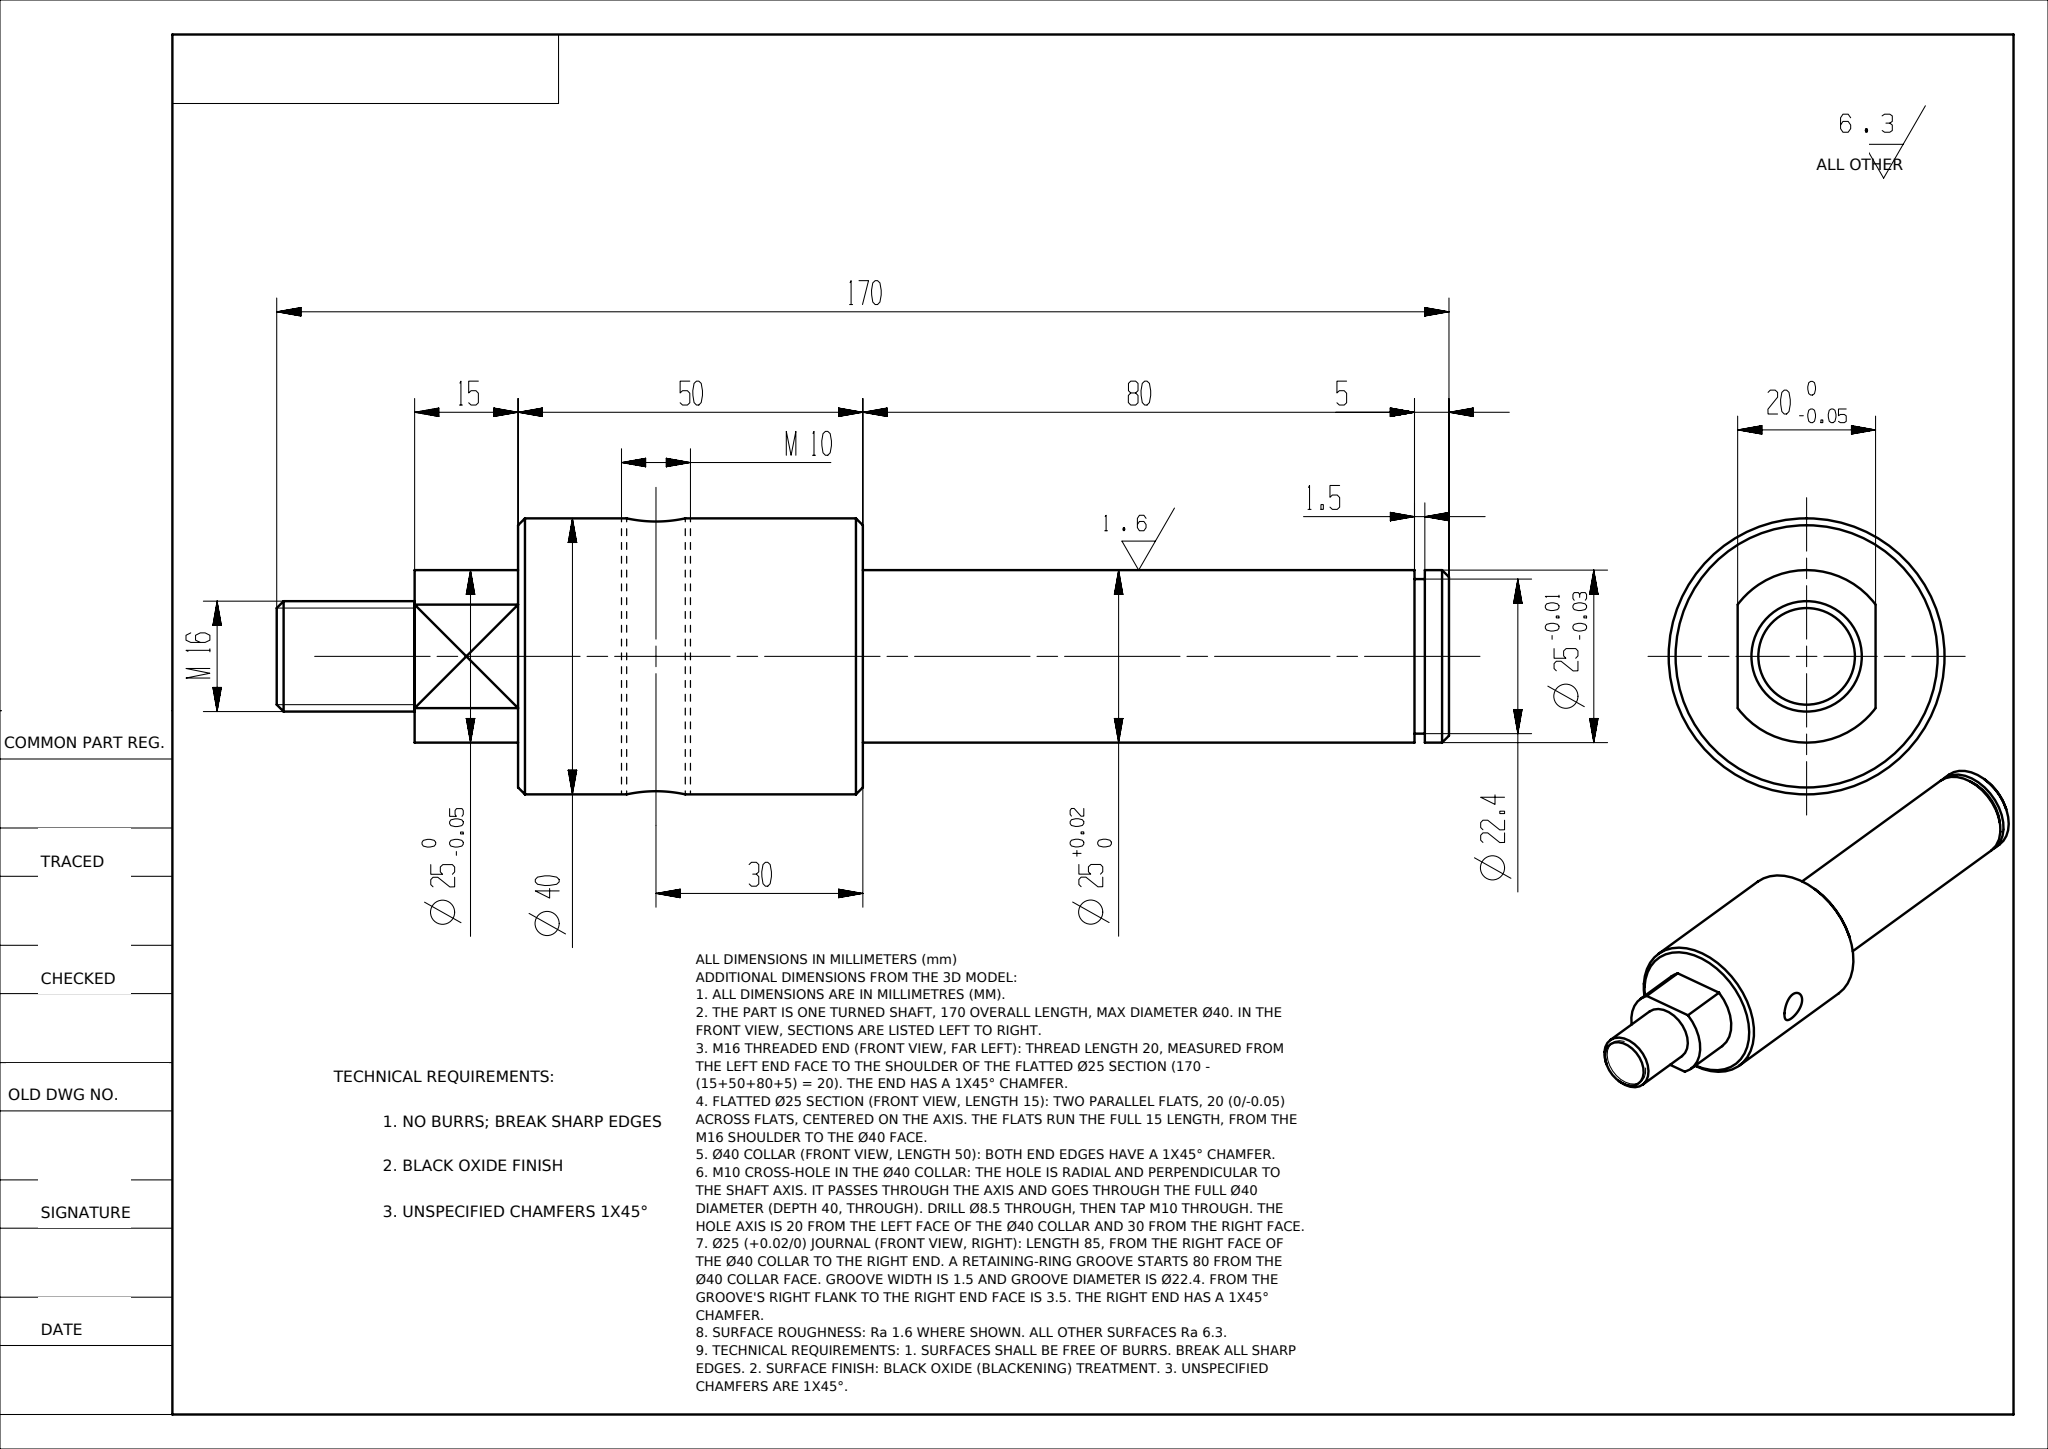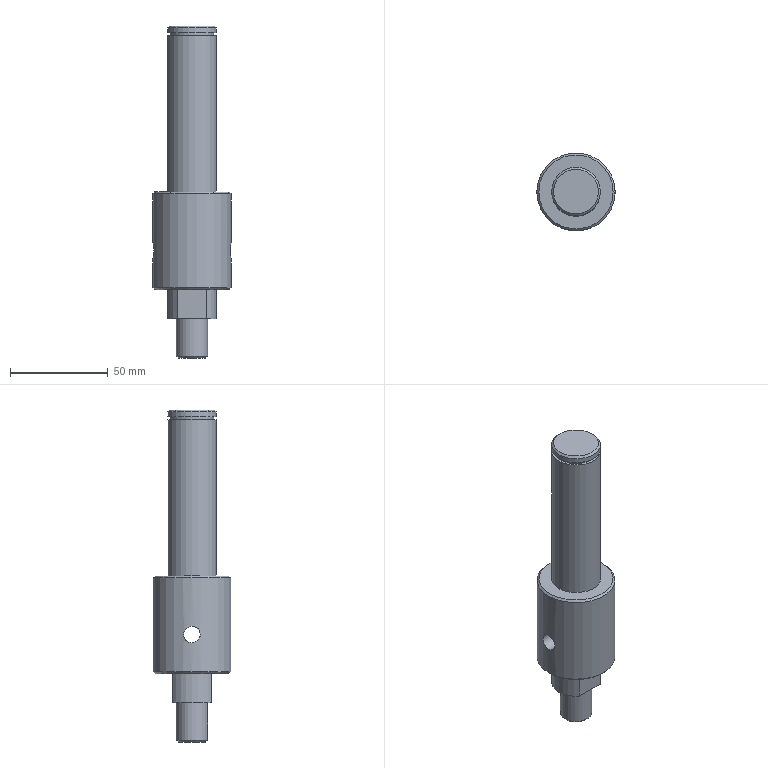Part | NX | mm | 1 solid | 21 faces | box 40 x 40 x 170 mm | volume 112586 mm3 | plane 9 | cylinder 8 | cone 4 | commonest cylinder face diameters 25 x4 40 x1 22.4 x1 16 x1 8.5 x1
STEP:
#1=CARTESIAN_POINT('',(0.,0.,0.));
#2=DIRECTION('',(0.,0.,1.));
#3=DIRECTION('',(1.,0.,0.));
#4=AXIS2_PLACEMENT_3D('',#1,#2,#3);
#5=(LENGTH_UNIT()NAMED_UNIT(*)SI_UNIT(.MILLI.,.METRE.));
#6=UNCERTAINTY_MEASURE_WITH_UNIT(LENGTH_MEASURE(0.0508),#5,'','');
#7=(NAMED_UNIT(*)PLANE_ANGLE_UNIT()SI_UNIT($,.RADIAN.));
#8=PLANE_ANGLE_MEASURE_WITH_UNIT(PLANE_ANGLE_MEASURE(0.01745),#7);
#9=DIMENSIONAL_EXPONENTS(0.,0.,0.,0.,0.,0.,0.);
#10=(CONVERSION_BASED_UNIT('',#8)NAMED_UNIT(#9)PLANE_ANGLE_UNIT());
#11=(NAMED_UNIT(*)SI_UNIT($,.STERADIAN.)SOLID_ANGLE_UNIT());
#12=(GEOMETRIC_REPRESENTATION_CONTEXT(3)GLOBAL_UNCERTAINTY_ASSIGNED_CONTEXT((#6))GLOBAL_UNIT_ASSIGNED_CONTEXT((#5,#10,#11))REPRESENTATION_CONTEXT('',''));
#13=SHAPE_REPRESENTATION('',(#4),#12);
#14=CARTESIAN_POINT('',(-7.5,10.,-15.));
#15=VERTEX_POINT('',#14);
#16=CARTESIAN_POINT('',(-7.5,10.,0.));
#17=VERTEX_POINT('',#16);
#18=CARTESIAN_POINT('',(-7.5,10.,0.));
#19=DIRECTION('',(0.,0.,1.));
#20=VECTOR('',#19,1.);
#21=LINE('',#18,#20);
#22=EDGE_CURVE('',#15,#17,#21,.T.);
#23=ORIENTED_EDGE('',*,*,#22,.F.);
#24=CARTESIAN_POINT('',(-7.5,-10.,-15.));
#25=VERTEX_POINT('',#24);
#26=CARTESIAN_POINT('',(0.,0.,-15.));
#27=DIRECTION('',(0.,0.,1.));
#28=DIRECTION('',(1.,0.,0.));
#29=AXIS2_PLACEMENT_3D('',#26,#27,#28);
#30=CIRCLE('',#29,12.5);
#31=EDGE_CURVE('',#15,#25,#30,.T.);
#32=ORIENTED_EDGE('',*,*,#31,.T.);
#33=CARTESIAN_POINT('',(-7.5,-10.,0.));
#34=VERTEX_POINT('',#33);
#35=CARTESIAN_POINT('',(-7.5,-10.,0.));
#36=DIRECTION('',(0.,0.,-1.));
#37=VECTOR('',#36,1.);
#38=LINE('',#35,#37);
#39=EDGE_CURVE('',#34,#25,#38,.T.);
#40=ORIENTED_EDGE('',*,*,#39,.F.);
#41=CARTESIAN_POINT('',(0.,0.,0.));
#42=DIRECTION('',(0.,0.,-1.));
#43=DIRECTION('',(-1.,0.,0.));
#44=AXIS2_PLACEMENT_3D('',#41,#42,#43);
#45=CIRCLE('',#44,12.5);
#46=EDGE_CURVE('',#34,#17,#45,.T.);
#47=ORIENTED_EDGE('',*,*,#46,.T.);
#48=EDGE_LOOP('',(#23,#32,#40,#47));
#49=FACE_OUTER_BOUND('',#48,.T.);
#50=CARTESIAN_POINT('',(0.,0.,0.));
#51=DIRECTION('',(0.,0.,-1.));
#52=DIRECTION('',(1.,0.,0.));
#53=AXIS2_PLACEMENT_3D('',#50,#51,#52);
#54=CYLINDRICAL_SURFACE('',#53,12.5);
#55=ADVANCED_FACE('',(#49),#54,.T.);
#56=CARTESIAN_POINT('',(12.5,0.,50.));
#57=VERTEX_POINT('',#56);
#58=CARTESIAN_POINT('',(0.,0.,50.));
#59=DIRECTION('',(0.,0.,1.));
#60=DIRECTION('',(1.,0.,0.));
#61=AXIS2_PLACEMENT_3D('',#58,#59,#60);
#62=CIRCLE('',#61,12.5);
#63=EDGE_CURVE('',#57,#57,#62,.T.);
#64=ORIENTED_EDGE('',*,*,#63,.T.);
#65=EDGE_LOOP('',(#64));
#66=FACE_BOUND('',#65,.T.);
#67=CARTESIAN_POINT('',(12.5,0.,130.));
#68=VERTEX_POINT('',#67);
#69=CARTESIAN_POINT('',(0.,0.,130.));
#70=DIRECTION('',(0.,0.,-1.));
#71=DIRECTION('',(1.,0.,0.));
#72=AXIS2_PLACEMENT_3D('',#69,#70,#71);
#73=CIRCLE('',#72,12.5);
#74=EDGE_CURVE('',#68,#68,#73,.T.);
#75=ORIENTED_EDGE('',*,*,#74,.T.);
#76=EDGE_LOOP('',(#75));
#77=FACE_BOUND('',#76,.T.);
#78=CARTESIAN_POINT('',(0.,0.,40.));
#79=DIRECTION('',(0.,0.,1.));
#80=DIRECTION('',(1.,0.,0.));
#81=AXIS2_PLACEMENT_3D('',#78,#79,#80);
#82=CYLINDRICAL_SURFACE('',#81,12.5);
#83=ADVANCED_FACE('',(#66,#77),#82,.T.);
#84=CARTESIAN_POINT('',(19.,0.,50.));
#85=VERTEX_POINT('',#84);
#86=CARTESIAN_POINT('',(0.,0.,50.));
#87=DIRECTION('',(0.,0.,1.));
#88=DIRECTION('',(1.,0.,0.));
#89=AXIS2_PLACEMENT_3D('',#86,#87,#88);
#90=CIRCLE('',#89,19.);
#91=EDGE_CURVE('',#85,#85,#90,.T.);
#92=ORIENTED_EDGE('',*,*,#91,.T.);
#93=EDGE_LOOP('',(#92));
#94=FACE_BOUND('',#93,.T.);
#95=ORIENTED_EDGE('',*,*,#63,.F.);
#96=EDGE_LOOP('',(#95));
#97=FACE_BOUND('',#96,.T.);
#98=CARTESIAN_POINT('',(0.,0.,50.));
#99=DIRECTION('',(0.,0.,1.));
#100=DIRECTION('',(1.,0.,0.));
#101=AXIS2_PLACEMENT_3D('',#98,#99,#100);
#102=PLANE('',#101);
#103=ADVANCED_FACE('',(#94,#97),#102,.T.);
#104=CARTESIAN_POINT('',(-19.,0.,0.));
#105=VERTEX_POINT('',#104);
#106=CARTESIAN_POINT('',(0.,0.,0.));
#107=DIRECTION('',(0.,0.,-1.));
#108=DIRECTION('',(-1.,0.,0.));
#109=AXIS2_PLACEMENT_3D('',#106,#107,#108);
#110=CIRCLE('',#109,19.);
#111=EDGE_CURVE('',#105,#105,#110,.T.);
#112=ORIENTED_EDGE('',*,*,#111,.T.);
#113=EDGE_LOOP('',(#112));
#114=FACE_BOUND('',#113,.T.);
#115=CARTESIAN_POINT('',(7.5,10.,0.));
#116=VERTEX_POINT('',#115);
#117=CARTESIAN_POINT('',(7.5,-10.,0.));
#118=VERTEX_POINT('',#117);
#119=CARTESIAN_POINT('',(0.,0.,0.));
#120=DIRECTION('',(0.,0.,-1.));
#121=DIRECTION('',(-1.,0.,0.));
#122=AXIS2_PLACEMENT_3D('',#119,#120,#121);
#123=CIRCLE('',#122,12.5);
#124=EDGE_CURVE('',#116,#118,#123,.T.);
#125=ORIENTED_EDGE('',*,*,#124,.F.);
#126=CARTESIAN_POINT('',(13.5,10.,0.));
#127=DIRECTION('',(-1.,0.,0.));
#128=VECTOR('',#127,1.);
#129=LINE('',#126,#128);
#130=EDGE_CURVE('',#116,#17,#129,.T.);
#131=ORIENTED_EDGE('',*,*,#130,.T.);
#132=ORIENTED_EDGE('',*,*,#46,.F.);
#133=CARTESIAN_POINT('',(-14.,-10.,0.));
#134=DIRECTION('',(1.,0.,0.));
#135=VECTOR('',#134,1.);
#136=LINE('',#133,#135);
#137=EDGE_CURVE('',#34,#118,#136,.T.);
#138=ORIENTED_EDGE('',*,*,#137,.T.);
#139=EDGE_LOOP('',(#125,#131,#132,#138));
#140=FACE_BOUND('',#139,.T.);
#141=CARTESIAN_POINT('',(0.,0.,0.));
#142=DIRECTION('',(0.,0.,-1.));
#143=DIRECTION('',(-1.,0.,0.));
#144=AXIS2_PLACEMENT_3D('',#141,#142,#143);
#145=PLANE('',#144);
#146=ADVANCED_FACE('',(#114,#140),#145,.T.);
#147=CARTESIAN_POINT('',(20.,0.,15.75));
#148=VERTEX_POINT('',#147);
#149=CARTESIAN_POINT('',(20.,0.,15.75));
#150=CARTESIAN_POINT('',(20.,0.4698,15.75));
#151=CARTESIAN_POINT('',(19.983,0.946,15.83));
#152=CARTESIAN_POINT('',(19.952,1.389,15.983));
#153=CARTESIAN_POINT('',(19.921,1.832,16.137));
#154=CARTESIAN_POINT('',(19.876,2.254,16.367));
#155=CARTESIAN_POINT('',(19.827,2.621,16.655));
#156=CARTESIAN_POINT('',(19.778,2.994,16.947));
#157=CARTESIAN_POINT('',(19.724,3.321,17.306));
#158=CARTESIAN_POINT('',(19.678,3.577,17.705));
#159=CARTESIAN_POINT('',(19.631,3.835,18.108));
#160=CARTESIAN_POINT('',(19.591,4.028,18.562));
#161=CARTESIAN_POINT('',(19.567,4.138,19.029));
#162=CARTESIAN_POINT('',(19.544,4.246,19.49));
#163=CARTESIAN_POINT('',(19.538,4.276,19.976));
#164=CARTESIAN_POINT('',(19.548,4.226,20.447));
#165=CARTESIAN_POINT('',(19.559,4.177,20.91));
#166=CARTESIAN_POINT('',(19.587,4.05,21.371));
#167=CARTESIAN_POINT('',(19.625,3.854,21.791));
#168=CARTESIAN_POINT('',(19.664,3.657,22.215));
#169=CARTESIAN_POINT('',(19.714,3.386,22.611));
#170=CARTESIAN_POINT('',(19.764,3.062,22.947));
#171=CARTESIAN_POINT('',(19.815,2.732,23.29));
#172=CARTESIAN_POINT('',(19.867,2.339,23.581));
#173=CARTESIAN_POINT('',(19.908,1.913,23.795));
#174=CARTESIAN_POINT('',(19.949,1.486,24.01));
#175=CARTESIAN_POINT('',(19.98,1.015,24.155));
#176=CARTESIAN_POINT('',(19.993,0.5393,24.216));
#177=CARTESIAN_POINT('',(20.005,0.07279,24.275));
#178=CARTESIAN_POINT('',(20.001,-0.411,24.256));
#179=CARTESIAN_POINT('',(19.981,-0.8711,24.16));
#180=CARTESIAN_POINT('',(19.961,-1.327,24.064));
#181=CARTESIAN_POINT('',(19.925,-1.771,23.891));
#182=CARTESIAN_POINT('',(19.882,-2.17,23.654));
#183=CARTESIAN_POINT('',(19.838,-2.574,23.414));
#184=CARTESIAN_POINT('',(19.785,-2.942,23.103));
#185=CARTESIAN_POINT('',(19.735,-3.245,22.744));
#186=CARTESIAN_POINT('',(19.684,-3.554,22.379));
#187=CARTESIAN_POINT('',(19.636,-3.803,21.956));
#188=CARTESIAN_POINT('',(19.601,-3.973,21.508));
#189=CARTESIAN_POINT('',(19.567,-4.142,21.063));
#190=CARTESIAN_POINT('',(19.546,-4.237,20.581));
#191=CARTESIAN_POINT('',(19.543,-4.249,20.103));
#192=CARTESIAN_POINT('',(19.541,-4.26,19.636));
#193=CARTESIAN_POINT('',(19.556,-4.192,19.16));
#194=CARTESIAN_POINT('',(19.585,-4.051,18.715));
#195=CARTESIAN_POINT('',(19.615,-3.91,18.271));
#196=CARTESIAN_POINT('',(19.658,-3.693,17.846));
#197=CARTESIAN_POINT('',(19.706,-3.417,17.473));
#198=CARTESIAN_POINT('',(19.755,-3.136,17.093));
#199=CARTESIAN_POINT('',(19.809,-2.787,16.756));
#200=CARTESIAN_POINT('',(19.856,-2.396,16.49));
#201=CARTESIAN_POINT('',(19.904,-2.001,16.22));
#202=CARTESIAN_POINT('',(19.945,-1.552,16.015));
#203=CARTESIAN_POINT('',(19.97,-1.088,15.892));
#204=CARTESIAN_POINT('',(19.99,-0.7349,15.798));
#205=CARTESIAN_POINT('',(20.,-0.3659,15.75));
#206=CARTESIAN_POINT('',(20.,0.,15.75));
#207=B_SPLINE_CURVE_WITH_KNOTS('',3,(#149,#150,#151,#152,#153,#154,#155,#156,#157,#158,#159,#160,#161,#162,#163,#164,#165,#166,#167,#168,#169,#170,#171,#172,#173,#174,#175,#176,#177,#178,#179,#180,#181,#182,#183,#184,#185,#186,#187,#188,#189,#190,#191,#192,#193,#194,#195,#196,#197,#198,#199,#200,#201,#202,#203,#204,#205,#206),.UNSPECIFIED.,.T.,.F.,(1,3,3,3,3,3,3,3,3,3,3,3,3,3,3,3,3,3,3,3,3,1),(-0.04096,0.,0.05289,0.1057,0.1593,0.2135,0.2668,0.3192,0.372,0.4259,0.4799,0.5329,0.5853,0.6384,0.6925,0.7463,0.7989,0.8514,0.9049,0.959,1.,1.053),.UNSPECIFIED.);
#208=EDGE_CURVE('',#148,#148,#207,.T.);
#209=ORIENTED_EDGE('',*,*,#208,.F.);
#210=EDGE_LOOP('',(#209));
#211=FACE_BOUND('',#210,.T.);
#212=CARTESIAN_POINT('',(-20.,0.,24.25));
#213=VERTEX_POINT('',#212);
#214=CARTESIAN_POINT('',(-20.,0.,24.25));
#215=CARTESIAN_POINT('',(-20.,0.4698,24.25));
#216=CARTESIAN_POINT('',(-19.983,0.946,24.17));
#217=CARTESIAN_POINT('',(-19.952,1.389,24.017));
#218=CARTESIAN_POINT('',(-19.921,1.832,23.863));
#219=CARTESIAN_POINT('',(-19.876,2.254,23.633));
#220=CARTESIAN_POINT('',(-19.827,2.621,23.345));
#221=CARTESIAN_POINT('',(-19.778,2.994,23.053));
#222=CARTESIAN_POINT('',(-19.724,3.321,22.694));
#223=CARTESIAN_POINT('',(-19.678,3.577,22.295));
#224=CARTESIAN_POINT('',(-19.631,3.835,21.892));
#225=CARTESIAN_POINT('',(-19.591,4.028,21.438));
#226=CARTESIAN_POINT('',(-19.567,4.138,20.971));
#227=CARTESIAN_POINT('',(-19.544,4.246,20.51));
#228=CARTESIAN_POINT('',(-19.538,4.276,20.024));
#229=CARTESIAN_POINT('',(-19.548,4.226,19.553));
#230=CARTESIAN_POINT('',(-19.559,4.177,19.09));
#231=CARTESIAN_POINT('',(-19.587,4.05,18.629));
#232=CARTESIAN_POINT('',(-19.625,3.854,18.209));
#233=CARTESIAN_POINT('',(-19.664,3.657,17.785));
#234=CARTESIAN_POINT('',(-19.714,3.386,17.389));
#235=CARTESIAN_POINT('',(-19.764,3.062,17.053));
#236=CARTESIAN_POINT('',(-19.815,2.732,16.71));
#237=CARTESIAN_POINT('',(-19.867,2.339,16.419));
#238=CARTESIAN_POINT('',(-19.908,1.913,16.205));
#239=CARTESIAN_POINT('',(-19.949,1.486,15.99));
#240=CARTESIAN_POINT('',(-19.98,1.015,15.845));
#241=CARTESIAN_POINT('',(-19.993,0.5393,15.784));
#242=CARTESIAN_POINT('',(-20.005,0.07279,15.725));
#243=CARTESIAN_POINT('',(-20.001,-0.411,15.744));
#244=CARTESIAN_POINT('',(-19.981,-0.8711,15.84));
#245=CARTESIAN_POINT('',(-19.961,-1.327,15.936));
#246=CARTESIAN_POINT('',(-19.925,-1.771,16.109));
#247=CARTESIAN_POINT('',(-19.882,-2.17,16.346));
#248=CARTESIAN_POINT('',(-19.838,-2.574,16.586));
#249=CARTESIAN_POINT('',(-19.785,-2.942,16.897));
#250=CARTESIAN_POINT('',(-19.735,-3.245,17.256));
#251=CARTESIAN_POINT('',(-19.684,-3.554,17.621));
#252=CARTESIAN_POINT('',(-19.636,-3.803,18.044));
#253=CARTESIAN_POINT('',(-19.601,-3.973,18.492));
#254=CARTESIAN_POINT('',(-19.567,-4.142,18.937));
#255=CARTESIAN_POINT('',(-19.546,-4.237,19.419));
#256=CARTESIAN_POINT('',(-19.543,-4.249,19.897));
#257=CARTESIAN_POINT('',(-19.541,-4.26,20.364));
#258=CARTESIAN_POINT('',(-19.556,-4.192,20.84));
#259=CARTESIAN_POINT('',(-19.585,-4.051,21.285));
#260=CARTESIAN_POINT('',(-19.615,-3.91,21.729));
#261=CARTESIAN_POINT('',(-19.658,-3.693,22.154));
#262=CARTESIAN_POINT('',(-19.706,-3.417,22.527));
#263=CARTESIAN_POINT('',(-19.755,-3.136,22.907));
#264=CARTESIAN_POINT('',(-19.809,-2.787,23.244));
#265=CARTESIAN_POINT('',(-19.856,-2.396,23.51));
#266=CARTESIAN_POINT('',(-19.904,-2.001,23.78));
#267=CARTESIAN_POINT('',(-19.945,-1.552,23.985));
#268=CARTESIAN_POINT('',(-19.97,-1.088,24.108));
#269=CARTESIAN_POINT('',(-19.99,-0.7349,24.202));
#270=CARTESIAN_POINT('',(-20.,-0.3659,24.25));
#271=CARTESIAN_POINT('',(-20.,0.,24.25));
#272=B_SPLINE_CURVE_WITH_KNOTS('',3,(#214,#215,#216,#217,#218,#219,#220,#221,#222,#223,#224,#225,#226,#227,#228,#229,#230,#231,#232,#233,#234,#235,#236,#237,#238,#239,#240,#241,#242,#243,#244,#245,#246,#247,#248,#249,#250,#251,#252,#253,#254,#255,#256,#257,#258,#259,#260,#261,#262,#263,#264,#265,#266,#267,#268,#269,#270,#271),.UNSPECIFIED.,.T.,.F.,(1,3,3,3,3,3,3,3,3,3,3,3,3,3,3,3,3,3,3,3,3,1),(-0.04096,0.,0.05289,0.1057,0.1593,0.2135,0.2668,0.3192,0.372,0.4259,0.4799,0.5329,0.5853,0.6384,0.6925,0.7463,0.7989,0.8514,0.9049,0.959,1.,1.053),.UNSPECIFIED.);
#273=EDGE_CURVE('',#213,#213,#272,.T.);
#274=ORIENTED_EDGE('',*,*,#273,.F.);
#275=EDGE_LOOP('',(#274));
#276=FACE_BOUND('',#275,.T.);
#277=CARTESIAN_POINT('',(-20.,0.,49.));
#278=VERTEX_POINT('',#277);
#279=CARTESIAN_POINT('',(0.,0.,49.));
#280=DIRECTION('',(0.,0.,-1.));
#281=DIRECTION('',(-1.,0.,0.));
#282=AXIS2_PLACEMENT_3D('',#279,#280,#281);
#283=CIRCLE('',#282,20.);
#284=EDGE_CURVE('',#278,#278,#283,.T.);
#285=ORIENTED_EDGE('',*,*,#284,.T.);
#286=EDGE_LOOP('',(#285));
#287=FACE_BOUND('',#286,.T.);
#288=CARTESIAN_POINT('',(-20.,0.,1.));
#289=VERTEX_POINT('',#288);
#290=CARTESIAN_POINT('',(0.,0.,1.));
#291=DIRECTION('',(0.,0.,1.));
#292=DIRECTION('',(-1.,0.,0.));
#293=AXIS2_PLACEMENT_3D('',#290,#291,#292);
#294=CIRCLE('',#293,20.);
#295=EDGE_CURVE('',#289,#289,#294,.T.);
#296=ORIENTED_EDGE('',*,*,#295,.T.);
#297=EDGE_LOOP('',(#296));
#298=FACE_BOUND('',#297,.T.);
#299=CARTESIAN_POINT('',(0.,0.,0.));
#300=DIRECTION('',(0.,0.,1.));
#301=DIRECTION('',(1.,0.,0.));
#302=AXIS2_PLACEMENT_3D('',#299,#300,#301);
#303=CYLINDRICAL_SURFACE('',#302,20.);
#304=ADVANCED_FACE('',(#211,#276,#287,#298),#303,.T.);
#305=CARTESIAN_POINT('',(11.2,0.,131.5));
#306=VERTEX_POINT('',#305);
#307=CARTESIAN_POINT('',(0.,0.,131.5));
#308=DIRECTION('',(0.,0.,-1.));
#309=DIRECTION('',(1.,0.,0.));
#310=AXIS2_PLACEMENT_3D('',#307,#308,#309);
#311=CIRCLE('',#310,11.2);
#312=EDGE_CURVE('',#306,#306,#311,.T.);
#313=ORIENTED_EDGE('',*,*,#312,.T.);
#314=EDGE_LOOP('',(#313));
#315=FACE_BOUND('',#314,.T.);
#316=CARTESIAN_POINT('',(11.2,0.,130.));
#317=VERTEX_POINT('',#316);
#318=CARTESIAN_POINT('',(0.,0.,130.));
#319=DIRECTION('',(0.,0.,-1.));
#320=DIRECTION('',(1.,0.,0.));
#321=AXIS2_PLACEMENT_3D('',#318,#319,#320);
#322=CIRCLE('',#321,11.2);
#323=EDGE_CURVE('',#317,#317,#322,.T.);
#324=ORIENTED_EDGE('',*,*,#323,.F.);
#325=EDGE_LOOP('',(#324));
#326=FACE_BOUND('',#325,.T.);
#327=CARTESIAN_POINT('',(0.,0.,100.75));
#328=DIRECTION('',(0.,0.,1.));
#329=DIRECTION('',(1.,0.,0.));
#330=AXIS2_PLACEMENT_3D('',#327,#328,#329);
#331=CYLINDRICAL_SURFACE('',#330,11.2);
#332=ADVANCED_FACE('',(#315,#326),#331,.T.);
#333=ORIENTED_EDGE('',*,*,#74,.F.);
#334=EDGE_LOOP('',(#333));
#335=FACE_BOUND('',#334,.T.);
#336=ORIENTED_EDGE('',*,*,#323,.T.);
#337=EDGE_LOOP('',(#336));
#338=FACE_BOUND('',#337,.T.);
#339=CARTESIAN_POINT('',(0.,0.,130.));
#340=DIRECTION('',(0.,0.,1.));
#341=DIRECTION('',(1.,0.,0.));
#342=AXIS2_PLACEMENT_3D('',#339,#340,#341);
#343=PLANE('',#342);
#344=ADVANCED_FACE('',(#335,#338),#343,.T.);
#345=CARTESIAN_POINT('',(12.5,0.,131.5));
#346=VERTEX_POINT('',#345);
#347=CARTESIAN_POINT('',(0.,0.,131.5));
#348=DIRECTION('',(0.,0.,-1.));
#349=DIRECTION('',(1.,0.,0.));
#350=AXIS2_PLACEMENT_3D('',#347,#348,#349);
#351=CIRCLE('',#350,12.5);
#352=EDGE_CURVE('',#346,#346,#351,.T.);
#353=ORIENTED_EDGE('',*,*,#352,.T.);
#354=EDGE_LOOP('',(#353));
#355=FACE_BOUND('',#354,.T.);
#356=ORIENTED_EDGE('',*,*,#312,.F.);
#357=EDGE_LOOP('',(#356));
#358=FACE_BOUND('',#357,.T.);
#359=CARTESIAN_POINT('',(0.,0.,131.5));
#360=DIRECTION('',(0.,0.,1.));
#361=DIRECTION('',(1.,0.,0.));
#362=AXIS2_PLACEMENT_3D('',#359,#360,#361);
#363=PLANE('',#362);
#364=ADVANCED_FACE('',(#355,#358),#363,.F.);
#365=CARTESIAN_POINT('',(11.5,0.,135.));
#366=VERTEX_POINT('',#365);
#367=CARTESIAN_POINT('',(0.,0.,135.));
#368=DIRECTION('',(0.,0.,1.));
#369=DIRECTION('',(1.,0.,0.));
#370=AXIS2_PLACEMENT_3D('',#367,#368,#369);
#371=CIRCLE('',#370,11.5);
#372=EDGE_CURVE('',#366,#366,#371,.T.);
#373=ORIENTED_EDGE('',*,*,#372,.T.);
#374=EDGE_LOOP('',(#373));
#375=FACE_OUTER_BOUND('',#374,.T.);
#376=CARTESIAN_POINT('',(0.,0.,135.));
#377=DIRECTION('',(0.,0.,1.));
#378=DIRECTION('',(1.,0.,0.));
#379=AXIS2_PLACEMENT_3D('',#376,#377,#378);
#380=PLANE('',#379);
#381=ADVANCED_FACE('',(#375),#380,.T.);
#382=CARTESIAN_POINT('',(-12.5,0.,134.));
#383=VERTEX_POINT('',#382);
#384=CARTESIAN_POINT('',(0.,0.,134.));
#385=DIRECTION('',(0.,0.,-1.));
#386=DIRECTION('',(-1.,0.,0.));
#387=AXIS2_PLACEMENT_3D('',#384,#385,#386);
#388=CIRCLE('',#387,12.5);
#389=EDGE_CURVE('',#383,#383,#388,.T.);
#390=ORIENTED_EDGE('',*,*,#389,.T.);
#391=EDGE_LOOP('',(#390));
#392=FACE_BOUND('',#391,.T.);
#393=ORIENTED_EDGE('',*,*,#352,.F.);
#394=EDGE_LOOP('',(#393));
#395=FACE_BOUND('',#394,.T.);
#396=CARTESIAN_POINT('',(0.,0.,40.));
#397=DIRECTION('',(0.,0.,1.));
#398=DIRECTION('',(1.,0.,0.));
#399=AXIS2_PLACEMENT_3D('',#396,#397,#398);
#400=CYLINDRICAL_SURFACE('',#399,12.5);
#401=ADVANCED_FACE('',(#392,#395),#400,.T.);
#402=CARTESIAN_POINT('',(7.5,-10.,-15.));
#403=VERTEX_POINT('',#402);
#404=CARTESIAN_POINT('',(-14.,-10.,-15.));
#405=DIRECTION('',(1.,0.,0.));
#406=VECTOR('',#405,1.);
#407=LINE('',#404,#406);
#408=EDGE_CURVE('',#25,#403,#407,.T.);
#409=ORIENTED_EDGE('',*,*,#408,.F.);
#410=ORIENTED_EDGE('',*,*,#31,.F.);
#411=CARTESIAN_POINT('',(7.5,10.,-15.));
#412=VERTEX_POINT('',#411);
#413=CARTESIAN_POINT('',(13.5,10.,-15.));
#414=DIRECTION('',(-1.,0.,0.));
#415=VECTOR('',#414,1.);
#416=LINE('',#413,#415);
#417=EDGE_CURVE('',#412,#15,#416,.T.);
#418=ORIENTED_EDGE('',*,*,#417,.F.);
#419=CARTESIAN_POINT('',(0.,0.,-15.));
#420=DIRECTION('',(0.,0.,1.));
#421=DIRECTION('',(1.,0.,0.));
#422=AXIS2_PLACEMENT_3D('',#419,#420,#421);
#423=CIRCLE('',#422,12.5);
#424=EDGE_CURVE('',#403,#412,#423,.T.);
#425=ORIENTED_EDGE('',*,*,#424,.F.);
#426=EDGE_LOOP('',(#409,#410,#418,#425));
#427=FACE_BOUND('',#426,.T.);
#428=CARTESIAN_POINT('',(-8.,0.,-15.));
#429=VERTEX_POINT('',#428);
#430=CARTESIAN_POINT('',(0.,0.,-15.));
#431=DIRECTION('',(0.,0.,-1.));
#432=DIRECTION('',(-1.,0.,0.));
#433=AXIS2_PLACEMENT_3D('',#430,#431,#432);
#434=CIRCLE('',#433,8.);
#435=EDGE_CURVE('',#429,#429,#434,.T.);
#436=ORIENTED_EDGE('',*,*,#435,.F.);
#437=EDGE_LOOP('',(#436));
#438=FACE_BOUND('',#437,.T.);
#439=CARTESIAN_POINT('',(0.,0.,-15.));
#440=DIRECTION('',(0.,0.,-1.));
#441=DIRECTION('',(-1.,0.,0.));
#442=AXIS2_PLACEMENT_3D('',#439,#440,#441);
#443=PLANE('',#442);
#444=ADVANCED_FACE('',(#427,#438),#443,.T.);
#445=CARTESIAN_POINT('',(7.5,10.,0.));
#446=DIRECTION('',(0.,0.,-1.));
#447=VECTOR('',#446,1.);
#448=LINE('',#445,#447);
#449=EDGE_CURVE('',#116,#412,#448,.T.);
#450=ORIENTED_EDGE('',*,*,#449,.F.);
#451=ORIENTED_EDGE('',*,*,#124,.T.);
#452=CARTESIAN_POINT('',(7.5,-10.,0.));
#453=DIRECTION('',(0.,0.,1.));
#454=VECTOR('',#453,1.);
#455=LINE('',#452,#454);
#456=EDGE_CURVE('',#403,#118,#455,.T.);
#457=ORIENTED_EDGE('',*,*,#456,.F.);
#458=ORIENTED_EDGE('',*,*,#424,.T.);
#459=EDGE_LOOP('',(#450,#451,#457,#458));
#460=FACE_OUTER_BOUND('',#459,.T.);
#461=CARTESIAN_POINT('',(0.,0.,0.));
#462=DIRECTION('',(0.,0.,-1.));
#463=DIRECTION('',(1.,0.,0.));
#464=AXIS2_PLACEMENT_3D('',#461,#462,#463);
#465=CYLINDRICAL_SURFACE('',#464,12.5);
#466=ADVANCED_FACE('',(#460),#465,.T.);
#467=CARTESIAN_POINT('',(-7.,0.,-35.));
#468=VERTEX_POINT('',#467);
#469=CARTESIAN_POINT('',(0.,0.,-35.));
#470=DIRECTION('',(0.,0.,-1.));
#471=DIRECTION('',(-1.,0.,0.));
#472=AXIS2_PLACEMENT_3D('',#469,#470,#471);
#473=CIRCLE('',#472,7.);
#474=EDGE_CURVE('',#468,#468,#473,.T.);
#475=ORIENTED_EDGE('',*,*,#474,.T.);
#476=EDGE_LOOP('',(#475));
#477=FACE_OUTER_BOUND('',#476,.T.);
#478=CARTESIAN_POINT('',(0.,0.,-35.));
#479=DIRECTION('',(0.,0.,-1.));
#480=DIRECTION('',(-1.,0.,0.));
#481=AXIS2_PLACEMENT_3D('',#478,#479,#480);
#482=PLANE('',#481);
#483=ADVANCED_FACE('',(#477),#482,.T.);
#484=CARTESIAN_POINT('',(-8.,0.,-34.));
#485=VERTEX_POINT('',#484);
#486=CARTESIAN_POINT('',(0.,0.,-34.));
#487=DIRECTION('',(0.,0.,1.));
#488=DIRECTION('',(-1.,0.,0.));
#489=AXIS2_PLACEMENT_3D('',#486,#487,#488);
#490=CIRCLE('',#489,8.);
#491=EDGE_CURVE('',#485,#485,#490,.T.);
#492=ORIENTED_EDGE('',*,*,#491,.T.);
#493=EDGE_LOOP('',(#492));
#494=FACE_BOUND('',#493,.T.);
#495=ORIENTED_EDGE('',*,*,#435,.T.);
#496=EDGE_LOOP('',(#495));
#497=FACE_BOUND('',#496,.T.);
#498=CARTESIAN_POINT('',(0.,0.,-15.));
#499=DIRECTION('',(0.,0.,-1.));
#500=DIRECTION('',(1.,0.,0.));
#501=AXIS2_PLACEMENT_3D('',#498,#499,#500);
#502=CYLINDRICAL_SURFACE('',#501,8.);
#503=ADVANCED_FACE('',(#494,#497),#502,.T.);
#504=ORIENTED_EDGE('',*,*,#456,.T.);
#505=ORIENTED_EDGE('',*,*,#137,.F.);
#506=ORIENTED_EDGE('',*,*,#39,.T.);
#507=ORIENTED_EDGE('',*,*,#408,.T.);
#508=EDGE_LOOP('',(#504,#505,#506,#507));
#509=FACE_OUTER_BOUND('',#508,.T.);
#510=CARTESIAN_POINT('',(-14.,-10.,0.));
#511=DIRECTION('',(0.,1.,0.));
#512=DIRECTION('',(0.,0.,1.));
#513=AXIS2_PLACEMENT_3D('',#510,#511,#512);
#514=PLANE('',#513);
#515=ADVANCED_FACE('',(#509),#514,.F.);
#516=ORIENTED_EDGE('',*,*,#22,.T.);
#517=ORIENTED_EDGE('',*,*,#130,.F.);
#518=ORIENTED_EDGE('',*,*,#449,.T.);
#519=ORIENTED_EDGE('',*,*,#417,.T.);
#520=EDGE_LOOP('',(#516,#517,#518,#519));
#521=FACE_OUTER_BOUND('',#520,.T.);
#522=CARTESIAN_POINT('',(13.5,10.,0.));
#523=DIRECTION('',(-0.,-1.,0.));
#524=DIRECTION('',(1.,-0.,0.));
#525=AXIS2_PLACEMENT_3D('',#522,#523,#524);
#526=PLANE('',#525);
#527=ADVANCED_FACE('',(#521),#526,.F.);
#528=ORIENTED_EDGE('',*,*,#372,.F.);
#529=EDGE_LOOP('',(#528));
#530=FACE_BOUND('',#529,.T.);
#531=ORIENTED_EDGE('',*,*,#389,.F.);
#532=EDGE_LOOP('',(#531));
#533=FACE_BOUND('',#532,.T.);
#534=CARTESIAN_POINT('',(0.,0.,134.));
#535=DIRECTION('',(0.,0.,-1.));
#536=DIRECTION('',(-1.,0.,0.));
#537=AXIS2_PLACEMENT_3D('',#534,#535,#536);
#538=CONICAL_SURFACE('',#537,12.5,45.);
#539=ADVANCED_FACE('',(#530,#533),#538,.T.);
#540=ORIENTED_EDGE('',*,*,#91,.F.);
#541=EDGE_LOOP('',(#540));
#542=FACE_BOUND('',#541,.T.);
#543=ORIENTED_EDGE('',*,*,#284,.F.);
#544=EDGE_LOOP('',(#543));
#545=FACE_BOUND('',#544,.T.);
#546=CARTESIAN_POINT('',(0.,0.,49.));
#547=DIRECTION('',(0.,0.,-1.));
#548=DIRECTION('',(-1.,0.,0.));
#549=AXIS2_PLACEMENT_3D('',#546,#547,#548);
#550=CONICAL_SURFACE('',#549,20.,45.);
#551=ADVANCED_FACE('',(#542,#545),#550,.T.);
#552=ORIENTED_EDGE('',*,*,#111,.F.);
#553=EDGE_LOOP('',(#552));
#554=FACE_BOUND('',#553,.T.);
#555=ORIENTED_EDGE('',*,*,#295,.F.);
#556=EDGE_LOOP('',(#555));
#557=FACE_BOUND('',#556,.T.);
#558=CARTESIAN_POINT('',(0.,0.,1.));
#559=DIRECTION('',(0.,0.,1.));
#560=DIRECTION('',(1.,0.,-0.));
#561=AXIS2_PLACEMENT_3D('',#558,#559,#560);
#562=CONICAL_SURFACE('',#561,20.,45.);
#563=ADVANCED_FACE('',(#554,#557),#562,.T.);
#564=ORIENTED_EDGE('',*,*,#474,.F.);
#565=EDGE_LOOP('',(#564));
#566=FACE_BOUND('',#565,.T.);
#567=ORIENTED_EDGE('',*,*,#491,.F.);
#568=EDGE_LOOP('',(#567));
#569=FACE_BOUND('',#568,.T.);
#570=CARTESIAN_POINT('',(0.,0.,-34.));
#571=DIRECTION('',(0.,0.,1.));
#572=DIRECTION('',(1.,0.,-0.));
#573=AXIS2_PLACEMENT_3D('',#570,#571,#572);
#574=CONICAL_SURFACE('',#573,8.,45.);
#575=ADVANCED_FACE('',(#566,#569),#574,.T.);
#576=ORIENTED_EDGE('',*,*,#208,.T.);
#577=EDGE_LOOP('',(#576));
#578=FACE_BOUND('',#577,.T.);
#579=ORIENTED_EDGE('',*,*,#273,.T.);
#580=EDGE_LOOP('',(#579));
#581=FACE_BOUND('',#580,.T.);
#582=CARTESIAN_POINT('',(20.,0.,20.));
#583=DIRECTION('',(-1.,0.,0.));
#584=DIRECTION('',(0.,0.,1.));
#585=AXIS2_PLACEMENT_3D('',#582,#583,#584);
#586=CYLINDRICAL_SURFACE('',#585,4.25);
#587=ADVANCED_FACE('',(#578,#581),#586,.F.);
#588=CLOSED_SHELL('',(#55,#83,#103,#146,#304,#332,#344,#364,#381,#401,#444,#466,#483,#503,#515,#527,#539,#551,#563,#575,#587));
#589=MANIFOLD_SOLID_BREP('',#588);
#590=ADVANCED_BREP_SHAPE_REPRESENTATION('',(#589),#12);
#591=SHAPE_REPRESENTATION_RELATIONSHIP('','',#13,#590);
#592=PRESENTATION_LAYER_ASSIGNMENT('','',(#589));
#593=COLOUR_RGB('',0.4,0.4,0.4);
#594=FILL_AREA_STYLE_COLOUR('',#593);
#595=FILL_AREA_STYLE('',(#594));
#596=SURFACE_STYLE_FILL_AREA(#595);
#597=SURFACE_SIDE_STYLE('',(#596));
#598=SURFACE_STYLE_USAGE(.BOTH.,#597);
#599=PRESENTATION_STYLE_ASSIGNMENT((#598));
#600=STYLED_ITEM('',(#599),#589);
#601=MECHANICAL_DESIGN_GEOMETRIC_PRESENTATION_REPRESENTATION('',(#600),#12);